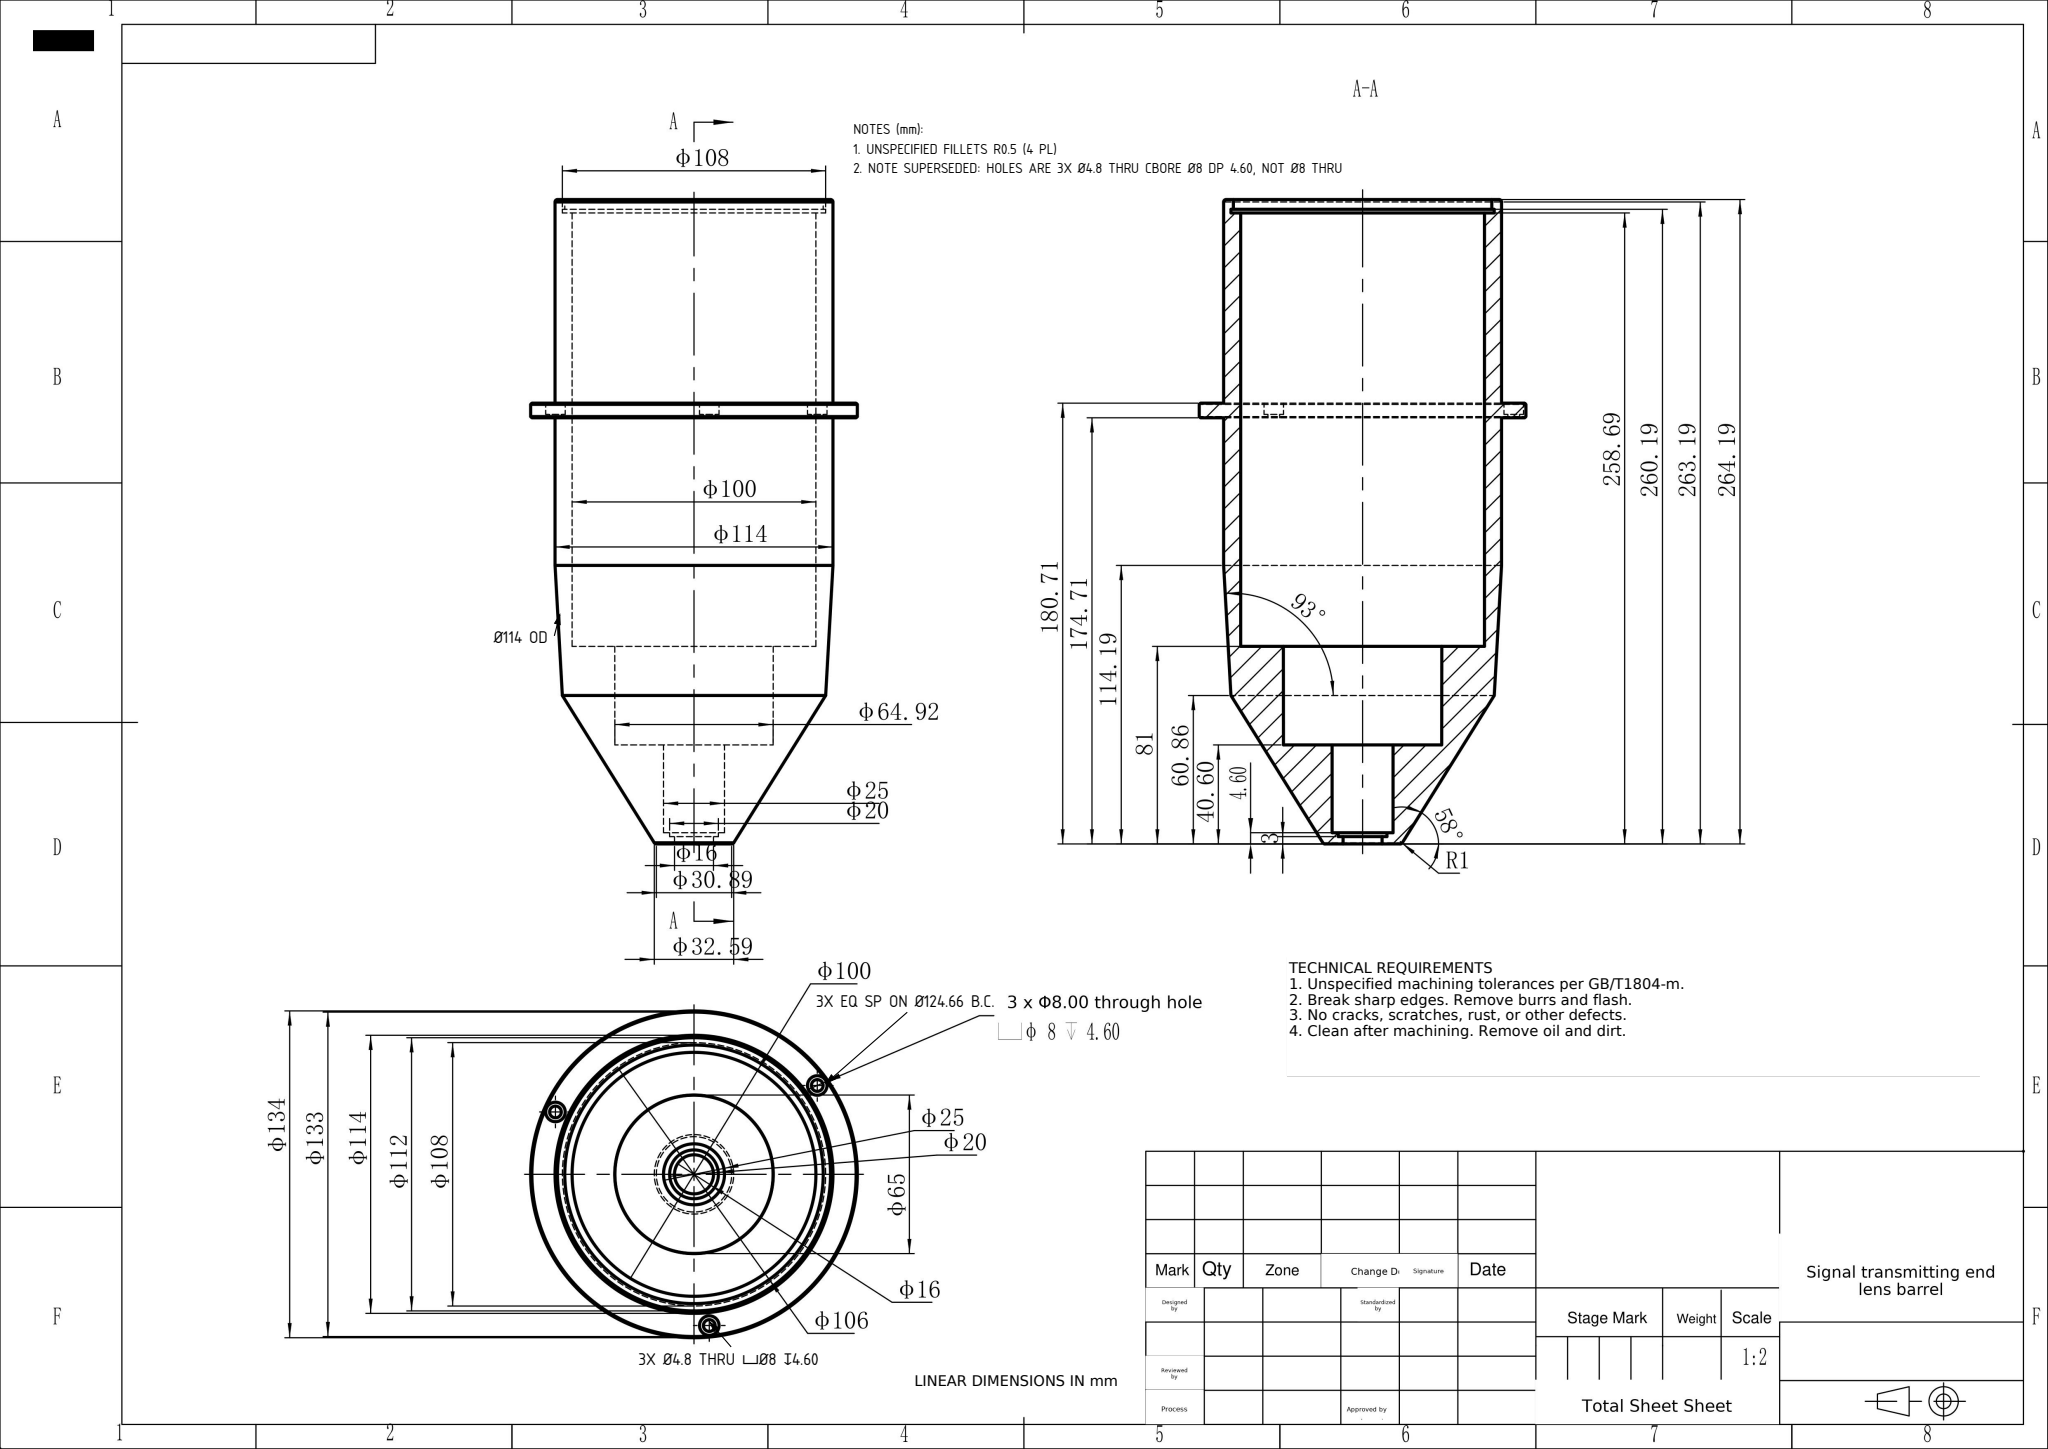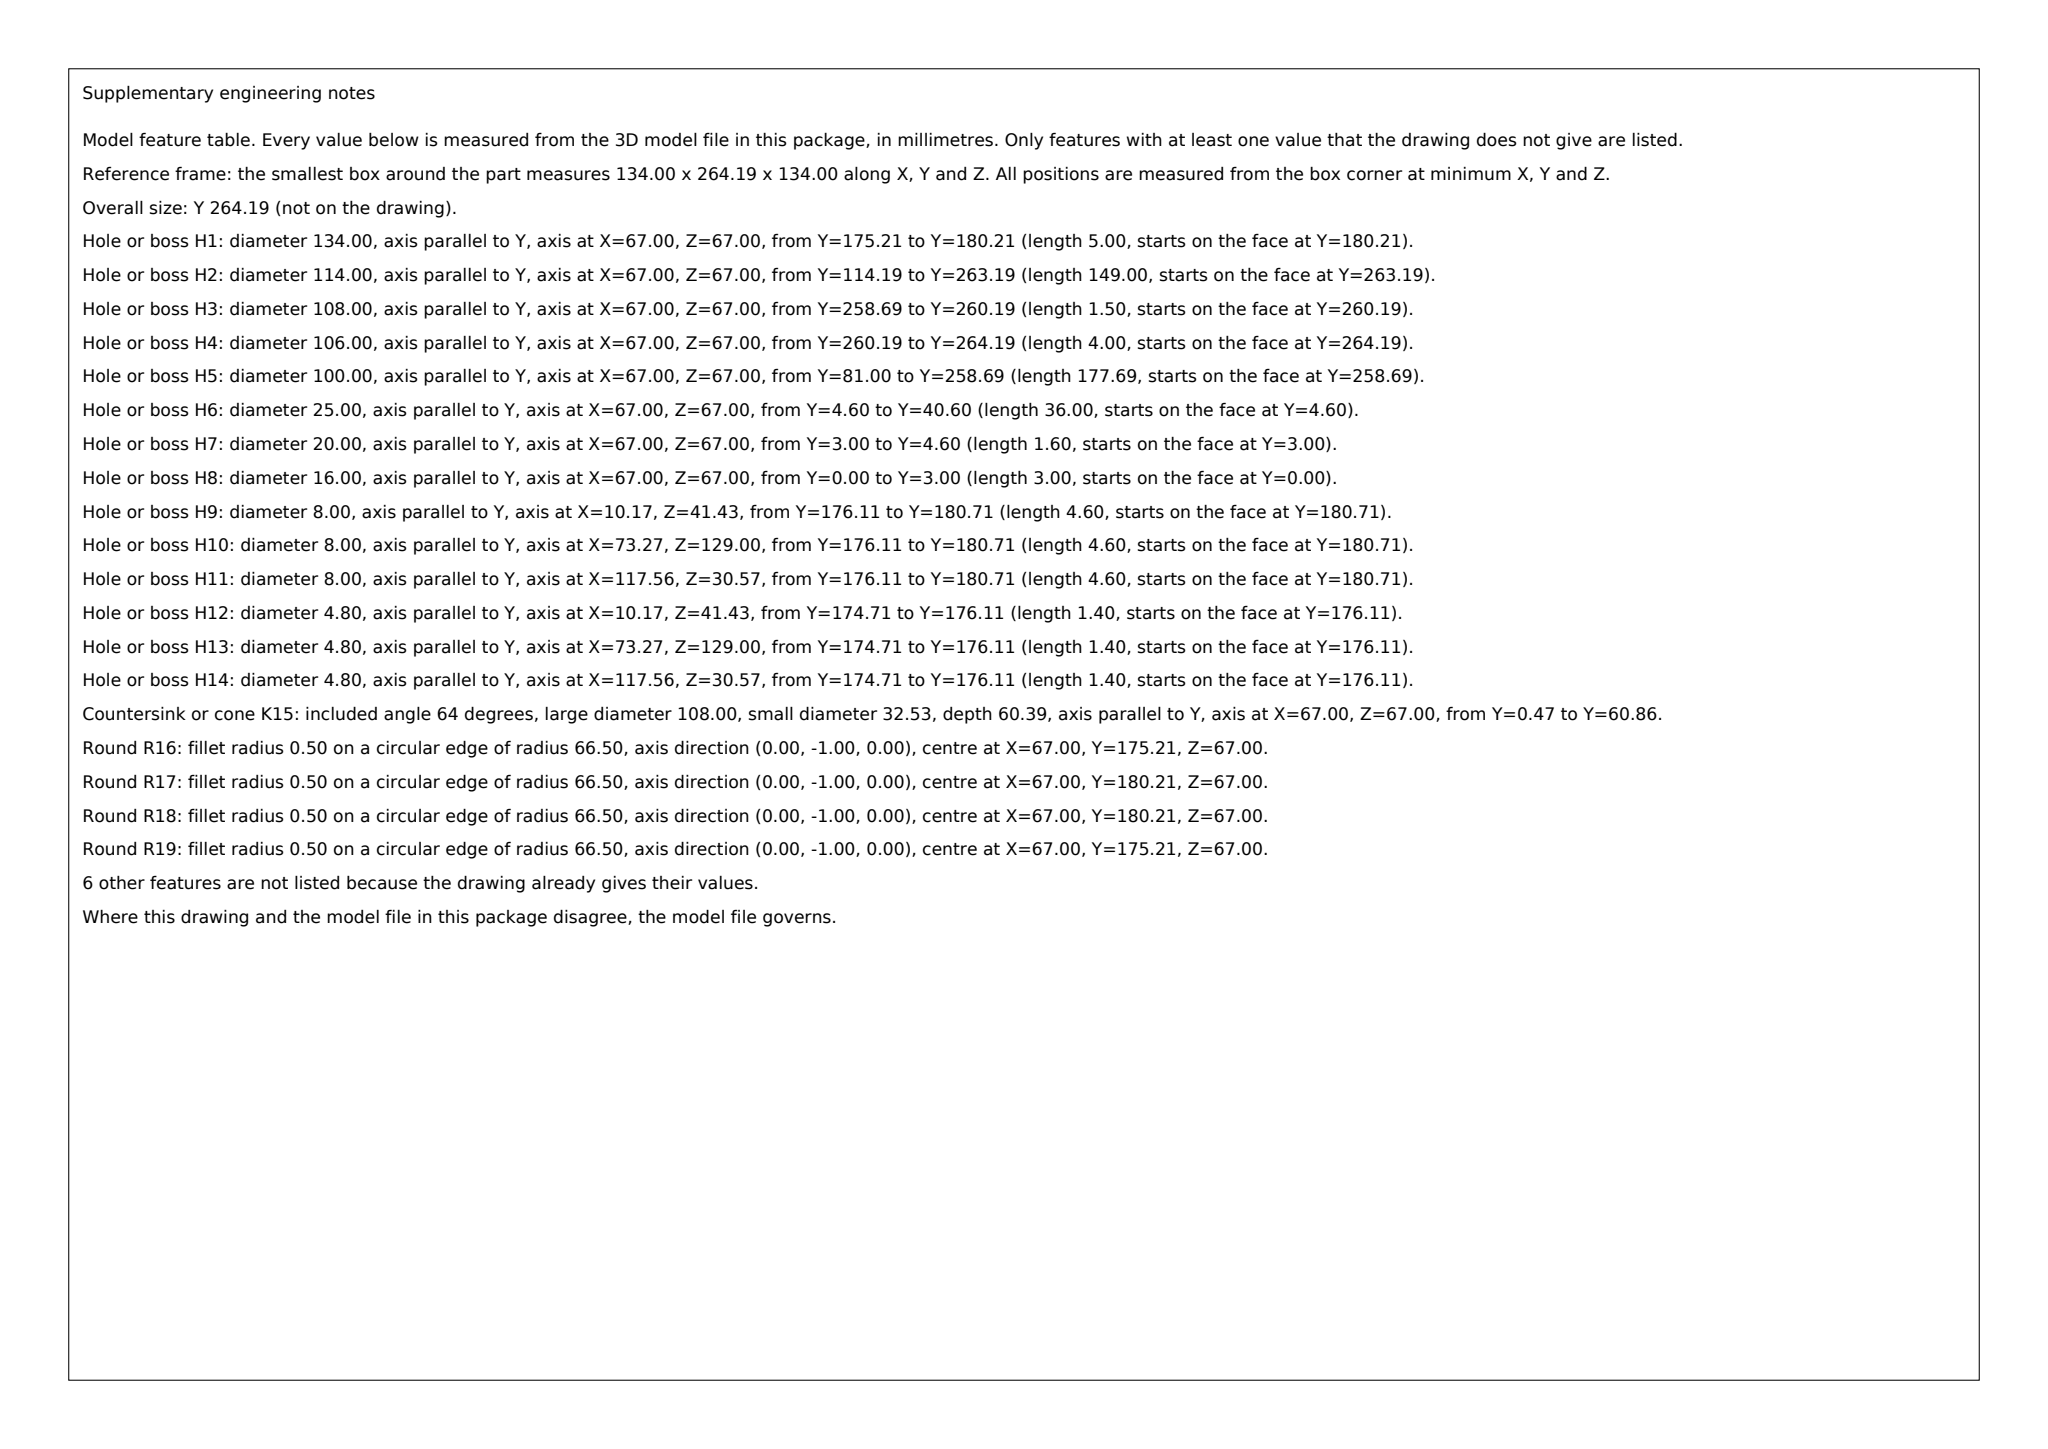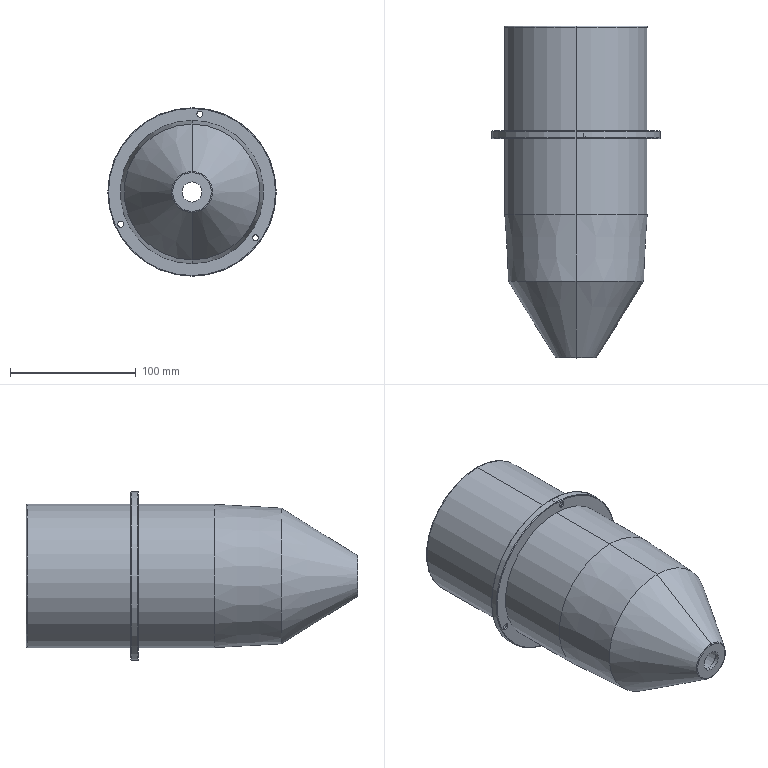Part | SolidWorks | mm | 1 solid | 57 faces | box 134 x 264.19 x 134 mm | volume 729677 mm3 | cylinder 30 | plane 13 | torus 8 | cone 6 | commonest cylinder face diameters 8 x6 4.8 x6 114 x4 134 x2 16 x2 20 x2 25 x2 100 x2
Drawing notes:
UNSPECIFIED FILLETS R0.5 (4 PL) | from the solid: fillet_radii [0.5,4] (plus [1.0,4] shown as R1)
Ø114 OD: 114.19 TO 174.71 & 180.71 TO 263.19; Ø112 = R1 TAN | from the solid: cyl [114,len 60.52] (174.71-60.52=114.19) and [114,len 82.48] (180.71+82.48=263.19); R1 fillets give 114-2=112
3X Ø4.8 THRU CBORE Ø8 DP 4.60 (C'BORE FROM FLANGE BTM FACE) | from the solid: Ø4.8 holes y174.7-176.1 (thru 6 thk flange), Ø8 c'bore y176.1-180.7 = 4.60 deep
3X Ø4.8 EQ SP ON Ø124.66 B.C., 1 HOLE 5.8° FROM VERT CL | from the solid: hole ctrs (123.1,36.1),(15.7,46.9),(78.8,134.5) about (72.5,72.5): R=62.33, angles 84.2/204.3/-35.7°
NOTE SUPERSEDED: HOLES ARE 3X Ø4.8 THRU CBORE Ø8 DP 4.60, NOT Ø8 THRU | from the solid: STEP: Ø4.8 thru y174.7-176.1 with Ø8 c'bore y176.1-180.7
build123d program:
from build123d import *

# Parameters (mm, degrees)
BOSS_EXTRUDE1_START                             = 6
SKETCH2_R                                       = 67
SKETCH2_R_2                                     = 57
BOSS_EXTRUDE1_DEPTH                             = 6
M4_HEX_SOCKET_HEAD_CAP_SCREW_CBORE1_D           = 4.8
M4_HEX_SOCKET_HEAD_CAP_SCREW_CBORE1_CBORE_D     = 8
M4_HEX_SOCKET_HEAD_CAP_SCREW_CBORE1_CBORE_DEPTH = 4.6
CIRPATTERN1_COUNT                               = 3
FILLET1_R                                       = 0.5
FILLET3_R                                       = 1


with BuildPart() as part:
    # Sketch1 → Revolve1 (revolve)
    with BuildSketch(Plane.XY, mode=Mode.PRIVATE) as revolve1_sk:
        Polygon((53, 23.481), (57, 23.481), (57, -126.519), (54, -179.852), (16, -240.709), (8, -240.709), (8, -237.709), (10, -237.709), (10, -236.113), (12.5, -236.113), (12.5, -200.113), (32.458, -200.113), (32.5, -159.709), (50, -159.709), (50, 17.981), (54, 17.981), (54, 19.481), (53, 19.481), align=None)
    revolve(revolve1_sk.sketch.rotate(Axis((0, -274.537, 0), (0, 1, 0)), 90), axis=Axis((0, -274.537, 0), (0, 1, 0)))

    # Sketch2 → Boss-Extrude1 (add)
    with BuildSketch(Plane.XZ.offset(60).offset(BOSS_EXTRUDE1_START)):
        with Locations(Location((0, 0, 0), (0, 0, 270))):
            Circle(SKETCH2_R)
        with Locations(Location((0, 0, 0), (0, 0, 270))):
            Circle(SKETCH2_R_2, mode=Mode.SUBTRACT)
    extrude(amount=-BOSS_EXTRUDE1_DEPTH)

    # M4 Hex Socket Head Cap Screw CBORE1 (through all)
    with Locations(Plane(origin=(0, -60, 0), x_dir=(1, 0, 0), z_dir=(0, 1, 0))):
        with Locations((6.267, -62)):
            m4_hex_socket_head_cap_screw_cbore1 = CounterBoreHole(M4_HEX_SOCKET_HEAD_CAP_SCREW_CBORE1_D / 2, M4_HEX_SOCKET_HEAD_CAP_SCREW_CBORE1_CBORE_D / 2, M4_HEX_SOCKET_HEAD_CAP_SCREW_CBORE1_CBORE_DEPTH)

    # CirPattern1: M4 Hex Socket Head Cap Screw CBORE1 ×3 about axis
    cirpattern1_axis = Axis((0, 0, 0), (0, 1, 0))
    for i in range(1, CIRPATTERN1_COUNT):
        add(m4_hex_socket_head_cap_screw_cbore1.rotate(cirpattern1_axis, i * 360 / CIRPATTERN1_COUNT), mode=Mode.SUBTRACT)

    # Fillet1
    fillet1_edges = [part.edges().sort_by_distance(p)[0] for p in [
        (0, -66, 67),
        (0, -60, 67),
    ]]
    fillet(fillet1_edges, radius=FILLET1_R)

    # Fillet3
    fillet3_edges = [part.edges().sort_by_distance(p)[0] for p in [
        (0, 23.481, 57),
        (0, -240.709, 16),
    ]]
    fillet(fillet3_edges, radius=FILLET3_R)


solid = part.part